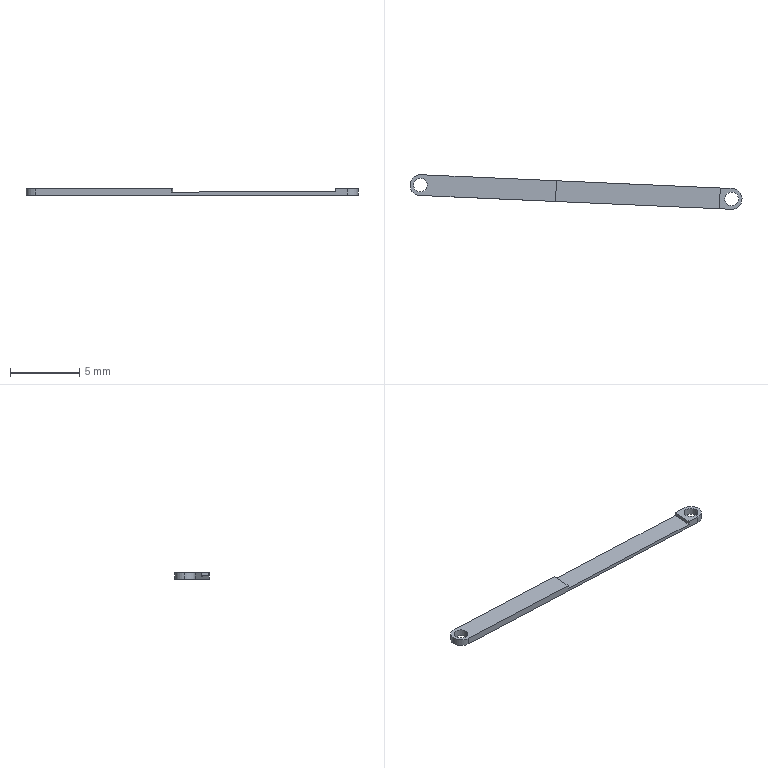Component | SolidWorks | Part1^Assembly1-1 | 1 solid | 15 faces | box 24 x 2.5 x 0.5 mm | volume 13 mm3 | plane 8 | cylinder 7 | commonest cylinder face diameters 1 x4 1.5 x3
STEP:
#1=CARTESIAN_POINT('',(0.368,-0.1082,0.3346));
#2=VERTEX_POINT('',#1);
#3=CARTESIAN_POINT('',(0.4073,-0.1104,0.3346));
#4=VERTEX_POINT('',#3);
#5=CARTESIAN_POINT('',(0.3877,-0.1093,0.3346));
#6=DIRECTION('',(-0.,0.,1.));
#7=DIRECTION('',(0.9983,-0.05778,0.));
#8=AXIS2_PLACEMENT_3D('',#5,#6,#7);
#9=CIRCLE('',#8,0.01969);
#10=EDGE_CURVE('',#2,#4,#9,.T.);
#11=ORIENTED_EDGE('',*,*,#10,.T.);
#12=CARTESIAN_POINT('',(0.4073,-0.1104,0.315));
#13=VERTEX_POINT('',#12);
#14=CARTESIAN_POINT('',(0.4073,-0.1104,0.3346));
#15=DIRECTION('',(0.,-0.,-1.));
#16=VECTOR('',#15,39.37);
#17=LINE('',#14,#16);
#18=EDGE_CURVE('',#4,#13,#17,.T.);
#19=ORIENTED_EDGE('',*,*,#18,.T.);
#20=CARTESIAN_POINT('',(0.368,-0.1082,0.315));
#21=VERTEX_POINT('',#20);
#22=CARTESIAN_POINT('',(0.3877,-0.1093,0.315));
#23=DIRECTION('',(-0.,0.,1.));
#24=DIRECTION('',(0.9983,-0.05778,0.));
#25=AXIS2_PLACEMENT_3D('',#22,#23,#24);
#26=CIRCLE('',#25,0.01969);
#27=EDGE_CURVE('',#21,#13,#26,.T.);
#28=ORIENTED_EDGE('',*,*,#27,.F.);
#29=CARTESIAN_POINT('',(0.368,-0.1082,0.3346));
#30=DIRECTION('',(0.,-0.,-1.));
#31=VECTOR('',#30,39.37);
#32=LINE('',#29,#31);
#33=EDGE_CURVE('',#2,#21,#32,.T.);
#34=ORIENTED_EDGE('',*,*,#33,.F.);
#35=EDGE_LOOP('',(#11,#19,#28,#34));
#36=FACE_OUTER_BOUND('',#35,.T.);
#37=CARTESIAN_POINT('',(0.3877,-0.1093,0.3346));
#38=DIRECTION('',(0.,-0.,-1.));
#39=DIRECTION('',(-0.9983,0.05778,0.));
#40=AXIS2_PLACEMENT_3D('',#37,#38,#39);
#41=CYLINDRICAL_SURFACE('',#40,0.01969);
#42=ADVANCED_FACE('',(#36),#41,.F.);
#43=CARTESIAN_POINT('',(-0.5178,-0.0688,0.3346));
#44=VERTEX_POINT('',#43);
#45=CARTESIAN_POINT('',(-0.4785,-0.07107,0.3346));
#46=VERTEX_POINT('',#45);
#47=CARTESIAN_POINT('',(-0.4982,-0.06993,0.3346));
#48=DIRECTION('',(-0.,0.,1.));
#49=DIRECTION('',(0.9983,-0.05778,0.));
#50=AXIS2_PLACEMENT_3D('',#47,#48,#49);
#51=CIRCLE('',#50,0.01969);
#52=EDGE_CURVE('',#44,#46,#51,.T.);
#53=ORIENTED_EDGE('',*,*,#52,.T.);
#54=CARTESIAN_POINT('',(-0.4785,-0.07107,0.315));
#55=VERTEX_POINT('',#54);
#56=CARTESIAN_POINT('',(-0.4785,-0.07107,0.3346));
#57=DIRECTION('',(0.,-0.,-1.));
#58=VECTOR('',#57,39.37);
#59=LINE('',#56,#58);
#60=EDGE_CURVE('',#46,#55,#59,.T.);
#61=ORIENTED_EDGE('',*,*,#60,.T.);
#62=CARTESIAN_POINT('',(-0.5178,-0.0688,0.315));
#63=VERTEX_POINT('',#62);
#64=CARTESIAN_POINT('',(-0.4982,-0.06993,0.315));
#65=DIRECTION('',(-0.,0.,1.));
#66=DIRECTION('',(0.9983,-0.05778,0.));
#67=AXIS2_PLACEMENT_3D('',#64,#65,#66);
#68=CIRCLE('',#67,0.01969);
#69=EDGE_CURVE('',#63,#55,#68,.T.);
#70=ORIENTED_EDGE('',*,*,#69,.F.);
#71=CARTESIAN_POINT('',(-0.5178,-0.0688,0.3346));
#72=DIRECTION('',(0.,-0.,-1.));
#73=VECTOR('',#72,39.37);
#74=LINE('',#71,#73);
#75=EDGE_CURVE('',#44,#63,#74,.T.);
#76=ORIENTED_EDGE('',*,*,#75,.F.);
#77=EDGE_LOOP('',(#53,#61,#70,#76));
#78=FACE_OUTER_BOUND('',#77,.T.);
#79=CARTESIAN_POINT('',(-0.4982,-0.06993,0.3346));
#80=DIRECTION('',(0.,-0.,-1.));
#81=DIRECTION('',(-0.9983,0.05778,0.));
#82=AXIS2_PLACEMENT_3D('',#79,#80,#81);
#83=CYLINDRICAL_SURFACE('',#82,0.01969);
#84=ADVANCED_FACE('',(#78),#83,.F.);
#85=CARTESIAN_POINT('',(-0.5276,-0.06823,0.3346));
#86=VERTEX_POINT('',#85);
#87=CARTESIAN_POINT('',(-0.4995,-0.09943,0.3346));
#88=VERTEX_POINT('',#87);
#89=CARTESIAN_POINT('',(-0.4982,-0.06993,0.3346));
#90=DIRECTION('',(-0.,0.,1.));
#91=DIRECTION('',(0.9983,-0.05778,0.));
#92=AXIS2_PLACEMENT_3D('',#89,#90,#91);
#93=CIRCLE('',#92,0.02953);
#94=EDGE_CURVE('',#86,#88,#93,.T.);
#95=ORIENTED_EDGE('',*,*,#94,.F.);
#96=CARTESIAN_POINT('',(-0.5276,-0.06823,0.315));
#97=VERTEX_POINT('',#96);
#98=CARTESIAN_POINT('',(-0.5276,-0.06823,0.3346));
#99=DIRECTION('',(0.,-0.,-1.));
#100=VECTOR('',#99,39.37);
#101=LINE('',#98,#100);
#102=EDGE_CURVE('',#86,#97,#101,.T.);
#103=ORIENTED_EDGE('',*,*,#102,.T.);
#104=CARTESIAN_POINT('',(-0.4995,-0.09943,0.315));
#105=VERTEX_POINT('',#104);
#106=CARTESIAN_POINT('',(-0.4982,-0.06993,0.315));
#107=DIRECTION('',(-0.,0.,1.));
#108=DIRECTION('',(0.9983,-0.05778,0.));
#109=AXIS2_PLACEMENT_3D('',#106,#107,#108);
#110=CIRCLE('',#109,0.02953);
#111=EDGE_CURVE('',#97,#105,#110,.T.);
#112=ORIENTED_EDGE('',*,*,#111,.T.);
#113=CARTESIAN_POINT('',(-0.4995,-0.09943,0.3346));
#114=DIRECTION('',(0.,-0.,-1.));
#115=VECTOR('',#114,39.37);
#116=LINE('',#113,#115);
#117=EDGE_CURVE('',#88,#105,#116,.T.);
#118=ORIENTED_EDGE('',*,*,#117,.F.);
#119=EDGE_LOOP('',(#95,#103,#112,#118));
#120=FACE_OUTER_BOUND('',#119,.T.);
#121=CARTESIAN_POINT('',(-0.4982,-0.06993,0.3346));
#122=DIRECTION('',(0.,-0.,-1.));
#123=DIRECTION('',(-0.9983,0.05778,0.));
#124=AXIS2_PLACEMENT_3D('',#121,#122,#123);
#125=CYLINDRICAL_SURFACE('',#124,0.02953);
#126=ADVANCED_FACE('',(#120),#125,.T.);
#127=CARTESIAN_POINT('',(-0.1106,-0.0576,0.3346));
#128=VERTEX_POINT('',#127);
#129=CARTESIAN_POINT('',(-0.114,-0.1166,0.3346));
#130=VERTEX_POINT('',#129);
#131=CARTESIAN_POINT('',(-0.1156,-0.1443,0.3346));
#132=DIRECTION('',(-0.05778,-0.9983,0.));
#133=VECTOR('',#132,39.37);
#134=LINE('',#131,#133);
#135=EDGE_CURVE('',#128,#130,#134,.T.);
#136=ORIENTED_EDGE('',*,*,#135,.F.);
#137=CARTESIAN_POINT('',(-0.4968,-0.04044,0.3346));
#138=VERTEX_POINT('',#137);
#139=CARTESIAN_POINT('',(-0.4968,-0.04044,0.3346));
#140=DIRECTION('',(-0.999,0.0444,-0.));
#141=VECTOR('',#140,39.37);
#142=LINE('',#139,#141);
#143=EDGE_CURVE('',#128,#138,#142,.T.);
#144=ORIENTED_EDGE('',*,*,#143,.T.);
#145=CARTESIAN_POINT('',(-0.4982,-0.06993,0.3346));
#146=DIRECTION('',(-0.,0.,1.));
#147=DIRECTION('',(0.9983,-0.05778,0.));
#148=AXIS2_PLACEMENT_3D('',#145,#146,#147);
#149=CIRCLE('',#148,0.02953);
#150=EDGE_CURVE('',#138,#86,#149,.T.);
#151=ORIENTED_EDGE('',*,*,#150,.T.);
#152=ORIENTED_EDGE('',*,*,#94,.T.);
#153=CARTESIAN_POINT('',(-0.4995,-0.09943,0.3346));
#154=DIRECTION('',(0.999,-0.0444,0.));
#155=VECTOR('',#154,39.37);
#156=LINE('',#153,#155);
#157=EDGE_CURVE('',#88,#130,#156,.T.);
#158=ORIENTED_EDGE('',*,*,#157,.T.);
#159=EDGE_LOOP('',(#136,#144,#151,#152,#158));
#160=FACE_OUTER_BOUND('',#159,.T.);
#161=ORIENTED_EDGE('',*,*,#52,.F.);
#162=CARTESIAN_POINT('',(-0.4982,-0.06993,0.3346));
#163=DIRECTION('',(-0.,0.,1.));
#164=DIRECTION('',(0.9983,-0.05778,0.));
#165=AXIS2_PLACEMENT_3D('',#162,#163,#164);
#166=CIRCLE('',#165,0.01969);
#167=EDGE_CURVE('',#46,#44,#166,.T.);
#168=ORIENTED_EDGE('',*,*,#167,.F.);
#169=EDGE_LOOP('',(#161,#168));
#170=FACE_BOUND('',#169,.T.);
#171=CARTESIAN_POINT('',(-0.4982,-0.06993,0.3346));
#172=DIRECTION('',(-0.,0.,1.));
#173=DIRECTION('',(0.9983,-0.05778,0.));
#174=AXIS2_PLACEMENT_3D('',#171,#172,#173);
#175=PLANE('',#174);
#176=ADVANCED_FACE('',(#160,#170),#175,.T.);
#177=CARTESIAN_POINT('',(0.3521,-0.1373,0.3346));
#178=VERTEX_POINT('',#177);
#179=CARTESIAN_POINT('',(0.3555,-0.07832,0.3346));
#180=VERTEX_POINT('',#179);
#181=CARTESIAN_POINT('',(0.3501,-0.1713,0.3346));
#182=DIRECTION('',(0.05778,0.9983,-0.));
#183=VECTOR('',#182,39.37);
#184=LINE('',#181,#183);
#185=EDGE_CURVE('',#178,#180,#184,.T.);
#186=ORIENTED_EDGE('',*,*,#185,.F.);
#187=CARTESIAN_POINT('',(0.3864,-0.1388,0.3346));
#188=VERTEX_POINT('',#187);
#189=CARTESIAN_POINT('',(-0.4995,-0.09943,0.3346));
#190=DIRECTION('',(0.999,-0.0444,0.));
#191=VECTOR('',#190,39.37);
#192=LINE('',#189,#191);
#193=EDGE_CURVE('',#178,#188,#192,.T.);
#194=ORIENTED_EDGE('',*,*,#193,.T.);
#195=CARTESIAN_POINT('',(0.389,-0.07981,0.3346));
#196=VERTEX_POINT('',#195);
#197=CARTESIAN_POINT('',(0.3877,-0.1093,0.3346));
#198=DIRECTION('',(-0.,0.,1.));
#199=DIRECTION('',(0.9983,-0.05778,0.));
#200=AXIS2_PLACEMENT_3D('',#197,#198,#199);
#201=CIRCLE('',#200,0.02953);
#202=EDGE_CURVE('',#188,#196,#201,.T.);
#203=ORIENTED_EDGE('',*,*,#202,.T.);
#204=CARTESIAN_POINT('',(-0.4968,-0.04044,0.3346));
#205=DIRECTION('',(-0.999,0.0444,-0.));
#206=VECTOR('',#205,39.37);
#207=LINE('',#204,#206);
#208=EDGE_CURVE('',#196,#180,#207,.T.);
#209=ORIENTED_EDGE('',*,*,#208,.T.);
#210=EDGE_LOOP('',(#186,#194,#203,#209));
#211=FACE_OUTER_BOUND('',#210,.T.);
#212=ORIENTED_EDGE('',*,*,#10,.F.);
#213=CARTESIAN_POINT('',(0.3877,-0.1093,0.3346));
#214=DIRECTION('',(-0.,0.,1.));
#215=DIRECTION('',(0.9983,-0.05778,0.));
#216=AXIS2_PLACEMENT_3D('',#213,#214,#215);
#217=CIRCLE('',#216,0.01969);
#218=EDGE_CURVE('',#4,#2,#217,.T.);
#219=ORIENTED_EDGE('',*,*,#218,.F.);
#220=EDGE_LOOP('',(#212,#219));
#221=FACE_BOUND('',#220,.T.);
#222=CARTESIAN_POINT('',(-0.4982,-0.06993,0.3346));
#223=DIRECTION('',(-0.,0.,1.));
#224=DIRECTION('',(0.9983,-0.05778,0.));
#225=AXIS2_PLACEMENT_3D('',#222,#223,#224);
#226=PLANE('',#225);
#227=ADVANCED_FACE('',(#211,#221),#226,.T.);
#228=CARTESIAN_POINT('',(-0.4968,-0.04044,0.315));
#229=VERTEX_POINT('',#228);
#230=CARTESIAN_POINT('',(-0.4982,-0.06993,0.315));
#231=DIRECTION('',(-0.,0.,1.));
#232=DIRECTION('',(0.9983,-0.05778,0.));
#233=AXIS2_PLACEMENT_3D('',#230,#231,#232);
#234=CIRCLE('',#233,0.02953);
#235=EDGE_CURVE('',#229,#97,#234,.T.);
#236=ORIENTED_EDGE('',*,*,#235,.F.);
#237=CARTESIAN_POINT('',(0.389,-0.07981,0.315));
#238=VERTEX_POINT('',#237);
#239=CARTESIAN_POINT('',(-0.4968,-0.04044,0.315));
#240=DIRECTION('',(-0.999,0.0444,-0.));
#241=VECTOR('',#240,39.37);
#242=LINE('',#239,#241);
#243=EDGE_CURVE('',#238,#229,#242,.T.);
#244=ORIENTED_EDGE('',*,*,#243,.F.);
#245=CARTESIAN_POINT('',(0.3864,-0.1388,0.315));
#246=VERTEX_POINT('',#245);
#247=CARTESIAN_POINT('',(0.3877,-0.1093,0.315));
#248=DIRECTION('',(-0.,0.,1.));
#249=DIRECTION('',(0.9983,-0.05778,0.));
#250=AXIS2_PLACEMENT_3D('',#247,#248,#249);
#251=CIRCLE('',#250,0.02953);
#252=EDGE_CURVE('',#246,#238,#251,.T.);
#253=ORIENTED_EDGE('',*,*,#252,.F.);
#254=CARTESIAN_POINT('',(-0.4995,-0.09943,0.315));
#255=DIRECTION('',(0.999,-0.0444,0.));
#256=VECTOR('',#255,39.37);
#257=LINE('',#254,#256);
#258=EDGE_CURVE('',#105,#246,#257,.T.);
#259=ORIENTED_EDGE('',*,*,#258,.F.);
#260=ORIENTED_EDGE('',*,*,#111,.F.);
#261=EDGE_LOOP('',(#236,#244,#253,#259,#260));
#262=FACE_OUTER_BOUND('',#261,.T.);
#263=ORIENTED_EDGE('',*,*,#69,.T.);
#264=CARTESIAN_POINT('',(-0.4982,-0.06993,0.315));
#265=DIRECTION('',(-0.,0.,1.));
#266=DIRECTION('',(0.9983,-0.05778,0.));
#267=AXIS2_PLACEMENT_3D('',#264,#265,#266);
#268=CIRCLE('',#267,0.01969);
#269=EDGE_CURVE('',#55,#63,#268,.T.);
#270=ORIENTED_EDGE('',*,*,#269,.T.);
#271=EDGE_LOOP('',(#263,#270));
#272=FACE_BOUND('',#271,.T.);
#273=ORIENTED_EDGE('',*,*,#27,.T.);
#274=CARTESIAN_POINT('',(0.3877,-0.1093,0.315));
#275=DIRECTION('',(-0.,0.,1.));
#276=DIRECTION('',(0.9983,-0.05778,0.));
#277=AXIS2_PLACEMENT_3D('',#274,#275,#276);
#278=CIRCLE('',#277,0.01969);
#279=EDGE_CURVE('',#13,#21,#278,.T.);
#280=ORIENTED_EDGE('',*,*,#279,.T.);
#281=EDGE_LOOP('',(#273,#280));
#282=FACE_BOUND('',#281,.T.);
#283=CARTESIAN_POINT('',(-0.4982,-0.06993,0.315));
#284=DIRECTION('',(-0.,0.,1.));
#285=DIRECTION('',(0.9983,-0.05778,0.));
#286=AXIS2_PLACEMENT_3D('',#283,#284,#285);
#287=PLANE('',#286);
#288=ADVANCED_FACE('',(#262,#272,#282),#287,.F.);
#289=ORIENTED_EDGE('',*,*,#102,.F.);
#290=ORIENTED_EDGE('',*,*,#150,.F.);
#291=CARTESIAN_POINT('',(-0.4968,-0.04044,0.3346));
#292=DIRECTION('',(0.,-0.,-1.));
#293=VECTOR('',#292,39.37);
#294=LINE('',#291,#293);
#295=EDGE_CURVE('',#138,#229,#294,.T.);
#296=ORIENTED_EDGE('',*,*,#295,.T.);
#297=ORIENTED_EDGE('',*,*,#235,.T.);
#298=EDGE_LOOP('',(#289,#290,#296,#297));
#299=FACE_OUTER_BOUND('',#298,.T.);
#300=CARTESIAN_POINT('',(-0.4982,-0.06993,0.3346));
#301=DIRECTION('',(0.,-0.,-1.));
#302=DIRECTION('',(-0.9983,0.05778,0.));
#303=AXIS2_PLACEMENT_3D('',#300,#301,#302);
#304=CYLINDRICAL_SURFACE('',#303,0.02953);
#305=ADVANCED_FACE('',(#299),#304,.T.);
#306=CARTESIAN_POINT('',(0.3521,-0.1373,0.3248));
#307=VERTEX_POINT('',#306);
#308=CARTESIAN_POINT('',(-0.114,-0.1166,0.3248));
#309=VERTEX_POINT('',#308);
#310=CARTESIAN_POINT('',(-0.4995,-0.09943,0.3248));
#311=DIRECTION('',(-0.999,0.0444,-0.));
#312=VECTOR('',#311,39.37);
#313=LINE('',#310,#312);
#314=EDGE_CURVE('',#307,#309,#313,.T.);
#315=ORIENTED_EDGE('',*,*,#314,.T.);
#316=CARTESIAN_POINT('',(-0.114,-0.1166,0.3346));
#317=DIRECTION('',(-0.,0.,1.));
#318=VECTOR('',#317,39.37);
#319=LINE('',#316,#318);
#320=EDGE_CURVE('',#309,#130,#319,.T.);
#321=ORIENTED_EDGE('',*,*,#320,.T.);
#322=ORIENTED_EDGE('',*,*,#157,.F.);
#323=ORIENTED_EDGE('',*,*,#117,.T.);
#324=ORIENTED_EDGE('',*,*,#258,.T.);
#325=CARTESIAN_POINT('',(0.3864,-0.1388,0.3346));
#326=DIRECTION('',(0.,-0.,-1.));
#327=VECTOR('',#326,39.37);
#328=LINE('',#325,#327);
#329=EDGE_CURVE('',#188,#246,#328,.T.);
#330=ORIENTED_EDGE('',*,*,#329,.F.);
#331=ORIENTED_EDGE('',*,*,#193,.F.);
#332=CARTESIAN_POINT('',(0.3521,-0.1373,0.3346));
#333=DIRECTION('',(0.,-0.,-1.));
#334=VECTOR('',#333,39.37);
#335=LINE('',#332,#334);
#336=EDGE_CURVE('',#178,#307,#335,.T.);
#337=ORIENTED_EDGE('',*,*,#336,.T.);
#338=EDGE_LOOP('',(#315,#321,#322,#323,#324,#330,#331,#337));
#339=FACE_OUTER_BOUND('',#338,.T.);
#340=CARTESIAN_POINT('',(-0.4995,-0.09943,0.3346));
#341=DIRECTION('',(0.0444,0.999,-0.));
#342=DIRECTION('',(-0.999,0.0444,-0.));
#343=AXIS2_PLACEMENT_3D('',#340,#341,#342);
#344=PLANE('',#343);
#345=ADVANCED_FACE('',(#339),#344,.F.);
#346=ORIENTED_EDGE('',*,*,#252,.T.);
#347=CARTESIAN_POINT('',(0.389,-0.07981,0.3346));
#348=DIRECTION('',(0.,-0.,-1.));
#349=VECTOR('',#348,39.37);
#350=LINE('',#347,#349);
#351=EDGE_CURVE('',#196,#238,#350,.T.);
#352=ORIENTED_EDGE('',*,*,#351,.F.);
#353=ORIENTED_EDGE('',*,*,#202,.F.);
#354=ORIENTED_EDGE('',*,*,#329,.T.);
#355=EDGE_LOOP('',(#346,#352,#353,#354));
#356=FACE_OUTER_BOUND('',#355,.T.);
#357=CARTESIAN_POINT('',(0.3877,-0.1093,0.3346));
#358=DIRECTION('',(0.,-0.,-1.));
#359=DIRECTION('',(-0.9983,0.05778,0.));
#360=AXIS2_PLACEMENT_3D('',#357,#358,#359);
#361=CYLINDRICAL_SURFACE('',#360,0.02953);
#362=ADVANCED_FACE('',(#356),#361,.T.);
#363=ORIENTED_EDGE('',*,*,#143,.F.);
#364=CARTESIAN_POINT('',(-0.1106,-0.0576,0.3248));
#365=VERTEX_POINT('',#364);
#366=CARTESIAN_POINT('',(-0.1106,-0.0576,0.3346));
#367=DIRECTION('',(0.,-0.,-1.));
#368=VECTOR('',#367,39.37);
#369=LINE('',#366,#368);
#370=EDGE_CURVE('',#128,#365,#369,.T.);
#371=ORIENTED_EDGE('',*,*,#370,.T.);
#372=CARTESIAN_POINT('',(0.3555,-0.07832,0.3248));
#373=VERTEX_POINT('',#372);
#374=CARTESIAN_POINT('',(-0.4968,-0.04044,0.3248));
#375=DIRECTION('',(0.999,-0.0444,0.));
#376=VECTOR('',#375,39.37);
#377=LINE('',#374,#376);
#378=EDGE_CURVE('',#365,#373,#377,.T.);
#379=ORIENTED_EDGE('',*,*,#378,.T.);
#380=CARTESIAN_POINT('',(0.3555,-0.07832,0.3346));
#381=DIRECTION('',(-0.,0.,1.));
#382=VECTOR('',#381,39.37);
#383=LINE('',#380,#382);
#384=EDGE_CURVE('',#373,#180,#383,.T.);
#385=ORIENTED_EDGE('',*,*,#384,.T.);
#386=ORIENTED_EDGE('',*,*,#208,.F.);
#387=ORIENTED_EDGE('',*,*,#351,.T.);
#388=ORIENTED_EDGE('',*,*,#243,.T.);
#389=ORIENTED_EDGE('',*,*,#295,.F.);
#390=EDGE_LOOP('',(#363,#371,#379,#385,#386,#387,#388,#389));
#391=FACE_OUTER_BOUND('',#390,.T.);
#392=CARTESIAN_POINT('',(-0.4968,-0.04044,0.3346));
#393=DIRECTION('',(-0.0444,-0.999,0.));
#394=DIRECTION('',(0.999,-0.0444,0.));
#395=AXIS2_PLACEMENT_3D('',#392,#393,#394);
#396=PLANE('',#395);
#397=ADVANCED_FACE('',(#391),#396,.F.);
#398=ORIENTED_EDGE('',*,*,#60,.F.);
#399=ORIENTED_EDGE('',*,*,#167,.T.);
#400=ORIENTED_EDGE('',*,*,#75,.T.);
#401=ORIENTED_EDGE('',*,*,#269,.F.);
#402=EDGE_LOOP('',(#398,#399,#400,#401));
#403=FACE_OUTER_BOUND('',#402,.T.);
#404=CARTESIAN_POINT('',(-0.4982,-0.06993,0.3346));
#405=DIRECTION('',(0.,-0.,-1.));
#406=DIRECTION('',(-0.9983,0.05778,0.));
#407=AXIS2_PLACEMENT_3D('',#404,#405,#406);
#408=CYLINDRICAL_SURFACE('',#407,0.01969);
#409=ADVANCED_FACE('',(#403),#408,.F.);
#410=ORIENTED_EDGE('',*,*,#18,.F.);
#411=ORIENTED_EDGE('',*,*,#218,.T.);
#412=ORIENTED_EDGE('',*,*,#33,.T.);
#413=ORIENTED_EDGE('',*,*,#279,.F.);
#414=EDGE_LOOP('',(#410,#411,#412,#413));
#415=FACE_OUTER_BOUND('',#414,.T.);
#416=CARTESIAN_POINT('',(0.3877,-0.1093,0.3346));
#417=DIRECTION('',(0.,-0.,-1.));
#418=DIRECTION('',(-0.9983,0.05778,0.));
#419=AXIS2_PLACEMENT_3D('',#416,#417,#418);
#420=CYLINDRICAL_SURFACE('',#419,0.01969);
#421=ADVANCED_FACE('',(#415),#420,.F.);
#422=CARTESIAN_POINT('',(-0.1156,-0.1443,0.3248));
#423=DIRECTION('',(-0.05778,-0.9983,0.));
#424=VECTOR('',#423,39.37);
#425=LINE('',#422,#424);
#426=EDGE_CURVE('',#365,#309,#425,.T.);
#427=ORIENTED_EDGE('',*,*,#426,.F.);
#428=ORIENTED_EDGE('',*,*,#370,.F.);
#429=ORIENTED_EDGE('',*,*,#135,.T.);
#430=ORIENTED_EDGE('',*,*,#320,.F.);
#431=EDGE_LOOP('',(#427,#428,#429,#430));
#432=FACE_OUTER_BOUND('',#431,.T.);
#433=CARTESIAN_POINT('',(-0.1156,-0.1443,0.3248));
#434=DIRECTION('',(-0.9983,0.05778,-0.));
#435=DIRECTION('',(-0.,0.,1.));
#436=AXIS2_PLACEMENT_3D('',#433,#434,#435);
#437=PLANE('',#436);
#438=ADVANCED_FACE('',(#432),#437,.F.);
#439=ORIENTED_EDGE('',*,*,#185,.T.);
#440=ORIENTED_EDGE('',*,*,#384,.F.);
#441=CARTESIAN_POINT('',(0.3501,-0.1713,0.3248));
#442=DIRECTION('',(0.05778,0.9983,-0.));
#443=VECTOR('',#442,39.37);
#444=LINE('',#441,#443);
#445=EDGE_CURVE('',#307,#373,#444,.T.);
#446=ORIENTED_EDGE('',*,*,#445,.F.);
#447=ORIENTED_EDGE('',*,*,#336,.F.);
#448=EDGE_LOOP('',(#439,#440,#446,#447));
#449=FACE_OUTER_BOUND('',#448,.T.);
#450=CARTESIAN_POINT('',(0.3501,-0.1713,0.3248));
#451=DIRECTION('',(0.9983,-0.05778,0.));
#452=DIRECTION('',(0.,-0.,-1.));
#453=AXIS2_PLACEMENT_3D('',#450,#451,#452);
#454=PLANE('',#453);
#455=ADVANCED_FACE('',(#449),#454,.F.);
#456=ORIENTED_EDGE('',*,*,#445,.T.);
#457=ORIENTED_EDGE('',*,*,#378,.F.);
#458=ORIENTED_EDGE('',*,*,#426,.T.);
#459=ORIENTED_EDGE('',*,*,#314,.F.);
#460=EDGE_LOOP('',(#456,#457,#458,#459));
#461=FACE_OUTER_BOUND('',#460,.T.);
#462=CARTESIAN_POINT('',(-0.2077,0.002977,0.3248));
#463=DIRECTION('',(0.,-0.,-1.));
#464=DIRECTION('',(-0.9983,0.05778,-0.));
#465=AXIS2_PLACEMENT_3D('',#462,#463,#464);
#466=PLANE('',#465);
#467=ADVANCED_FACE('',(#461),#466,.F.);
#468=CLOSED_SHELL('',(#42,#84,#126,#176,#227,#288,#305,#345,#362,#397,#409,#421,#438,#455,#467));
#469=MANIFOLD_SOLID_BREP('',#468);
#470=CARTESIAN_POINT('',(0.,0.,0.));
#471=DIRECTION('',(0.,0.,1.));
#472=DIRECTION('',(1.,0.,0.));
#473=AXIS2_PLACEMENT_3D('',#470,#471,#472);
#474=(LENGTH_UNIT()NAMED_UNIT(*)SI_UNIT($,.METRE.));
#475=LENGTH_MEASURE_WITH_UNIT(LENGTH_MEASURE(0.0254),#474);
#476=DIMENSIONAL_EXPONENTS(1.,0.,0.,0.,0.,0.,0.);
#477=(CONVERSION_BASED_UNIT('',#475)LENGTH_UNIT()NAMED_UNIT(#476));
#478=UNCERTAINTY_MEASURE_WITH_UNIT(LENGTH_MEASURE(0.00001),#477,'','');
#479=(NAMED_UNIT(*)PLANE_ANGLE_UNIT()SI_UNIT($,.RADIAN.));
#480=(NAMED_UNIT(*)SI_UNIT($,.STERADIAN.)SOLID_ANGLE_UNIT());
#481=(GEOMETRIC_REPRESENTATION_CONTEXT(3)GLOBAL_UNCERTAINTY_ASSIGNED_CONTEXT((#478))GLOBAL_UNIT_ASSIGNED_CONTEXT((#477,#479,#480))REPRESENTATION_CONTEXT('',''));
#482=ADVANCED_BREP_SHAPE_REPRESENTATION('',(#469,#473),#481);
#483=COLOUR_RGB('',0.7922,0.8196,0.9333);
#484=FILL_AREA_STYLE_COLOUR('',#483);
#485=FILL_AREA_STYLE('',(#484));
#486=SURFACE_STYLE_FILL_AREA(#485);
#487=SURFACE_SIDE_STYLE('',(#486));
#488=SURFACE_STYLE_USAGE(.BOTH.,#487);
#489=PRESENTATION_STYLE_ASSIGNMENT((#488));
#490=STYLED_ITEM('',(#489),#469);
#491=(LENGTH_UNIT()NAMED_UNIT(*)SI_UNIT($,.METRE.));
#492=LENGTH_MEASURE_WITH_UNIT(LENGTH_MEASURE(0.0254),#491);
#493=DIMENSIONAL_EXPONENTS(1.,0.,0.,0.,0.,0.,0.);
#494=(CONVERSION_BASED_UNIT('',#492)LENGTH_UNIT()NAMED_UNIT(#493));
#495=UNCERTAINTY_MEASURE_WITH_UNIT(LENGTH_MEASURE(0.00001),#494,'','');
#496=(NAMED_UNIT(*)PLANE_ANGLE_UNIT()SI_UNIT($,.RADIAN.));
#497=(NAMED_UNIT(*)SI_UNIT($,.STERADIAN.)SOLID_ANGLE_UNIT());
#498=(GEOMETRIC_REPRESENTATION_CONTEXT(3)GLOBAL_UNCERTAINTY_ASSIGNED_CONTEXT((#495))GLOBAL_UNIT_ASSIGNED_CONTEXT((#494,#496,#497))REPRESENTATION_CONTEXT('',''));
#499=MECHANICAL_DESIGN_GEOMETRIC_PRESENTATION_REPRESENTATION('',(#490),#498);
#500=PRESENTATION_LAYER_ASSIGNMENT('','',(#490));